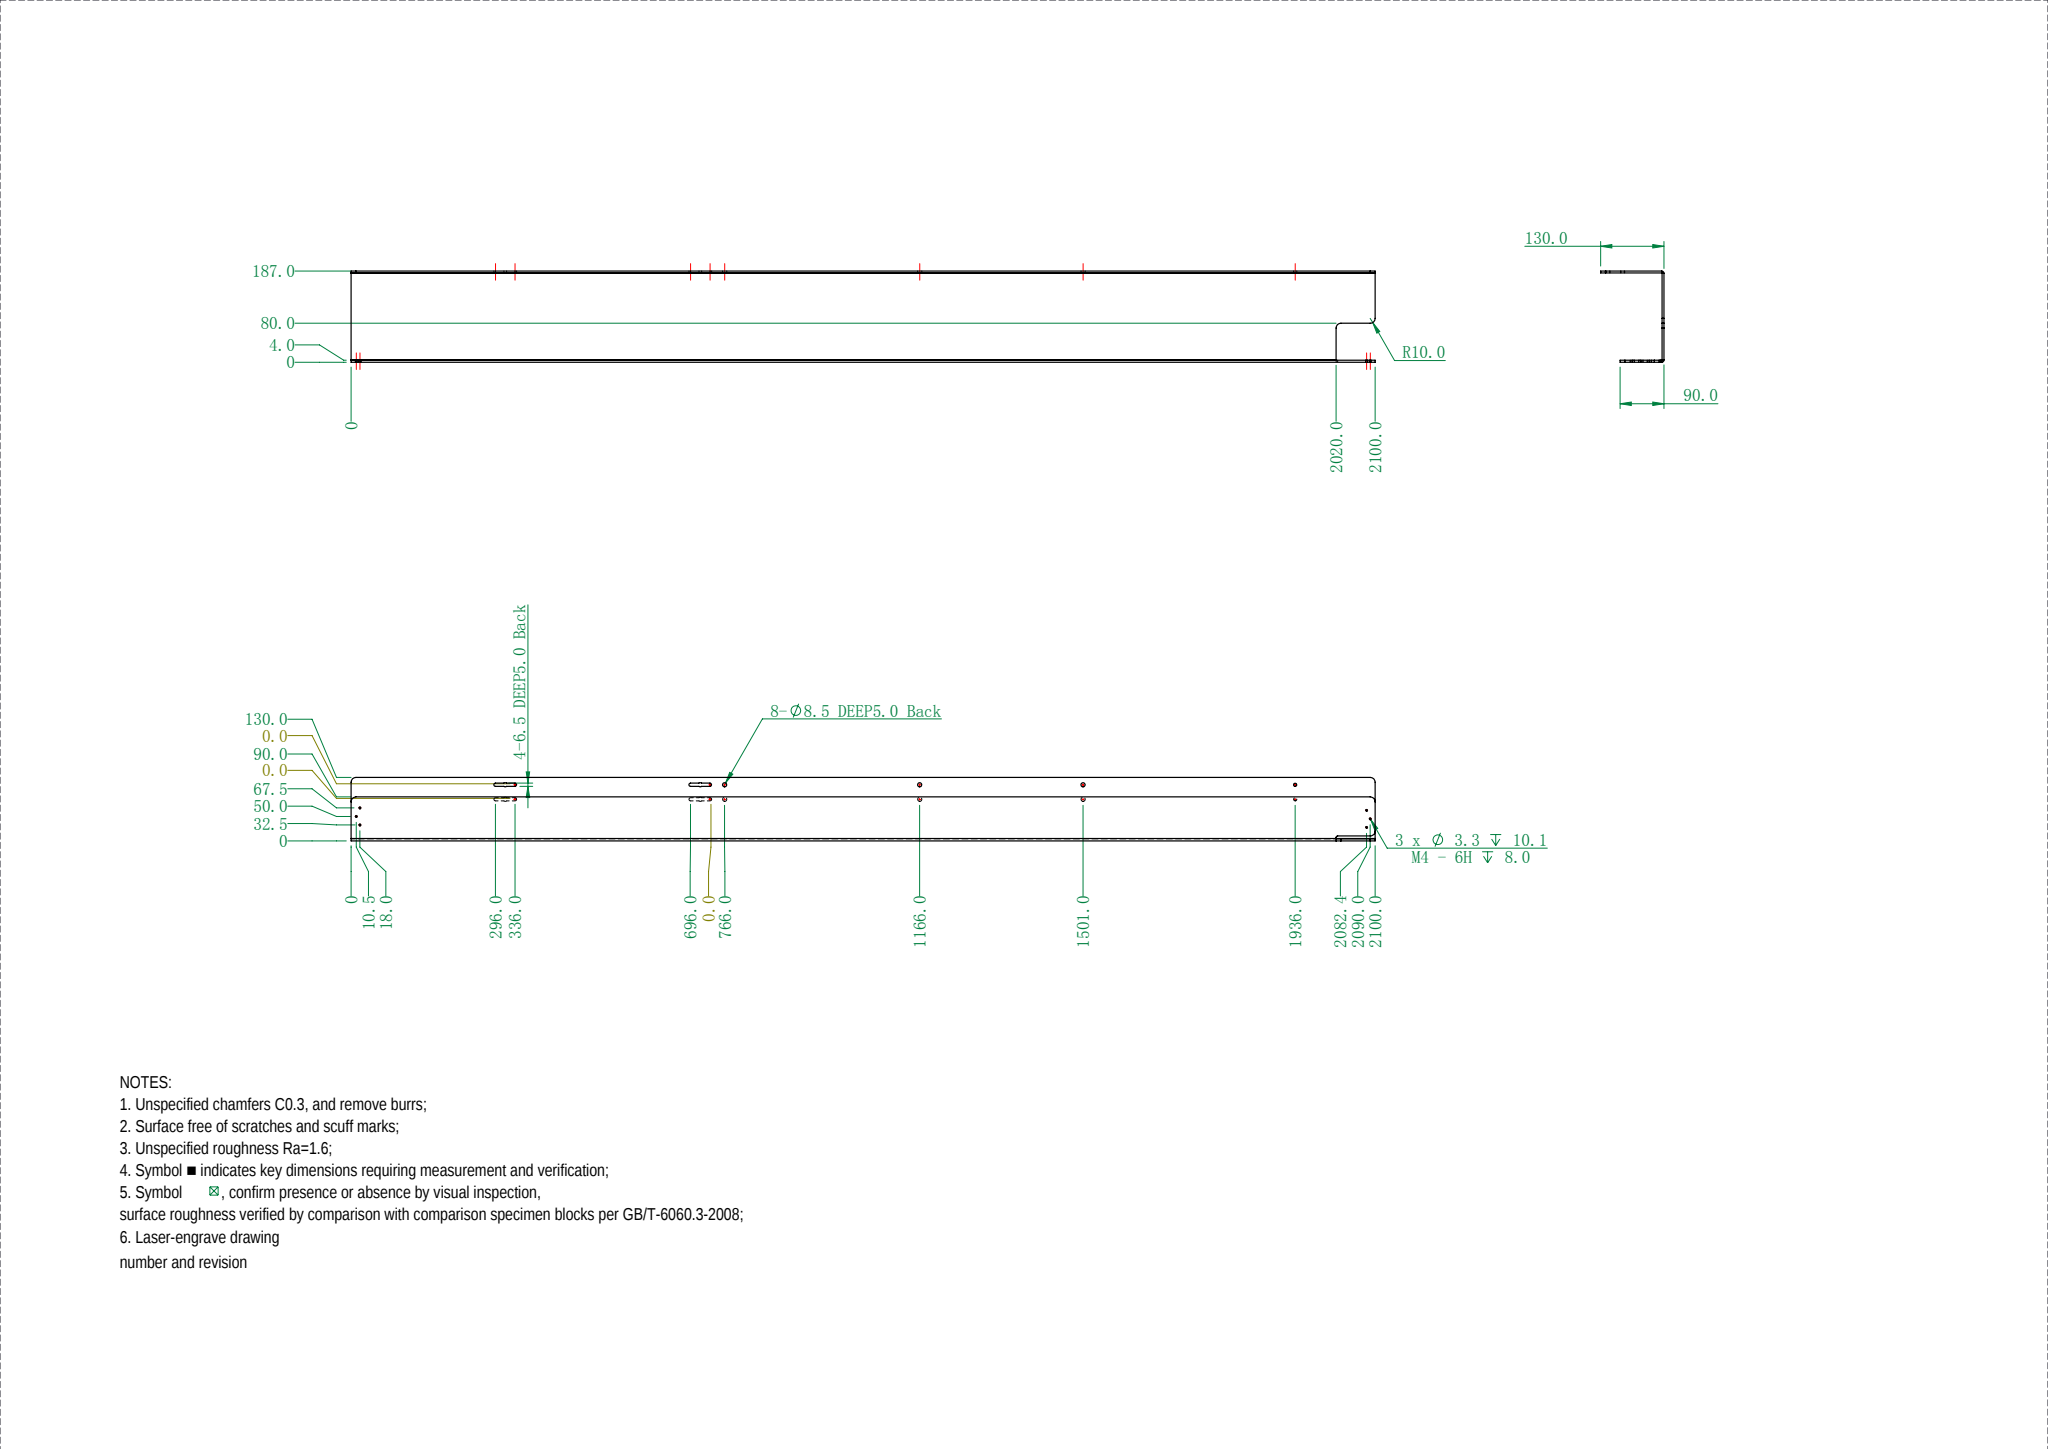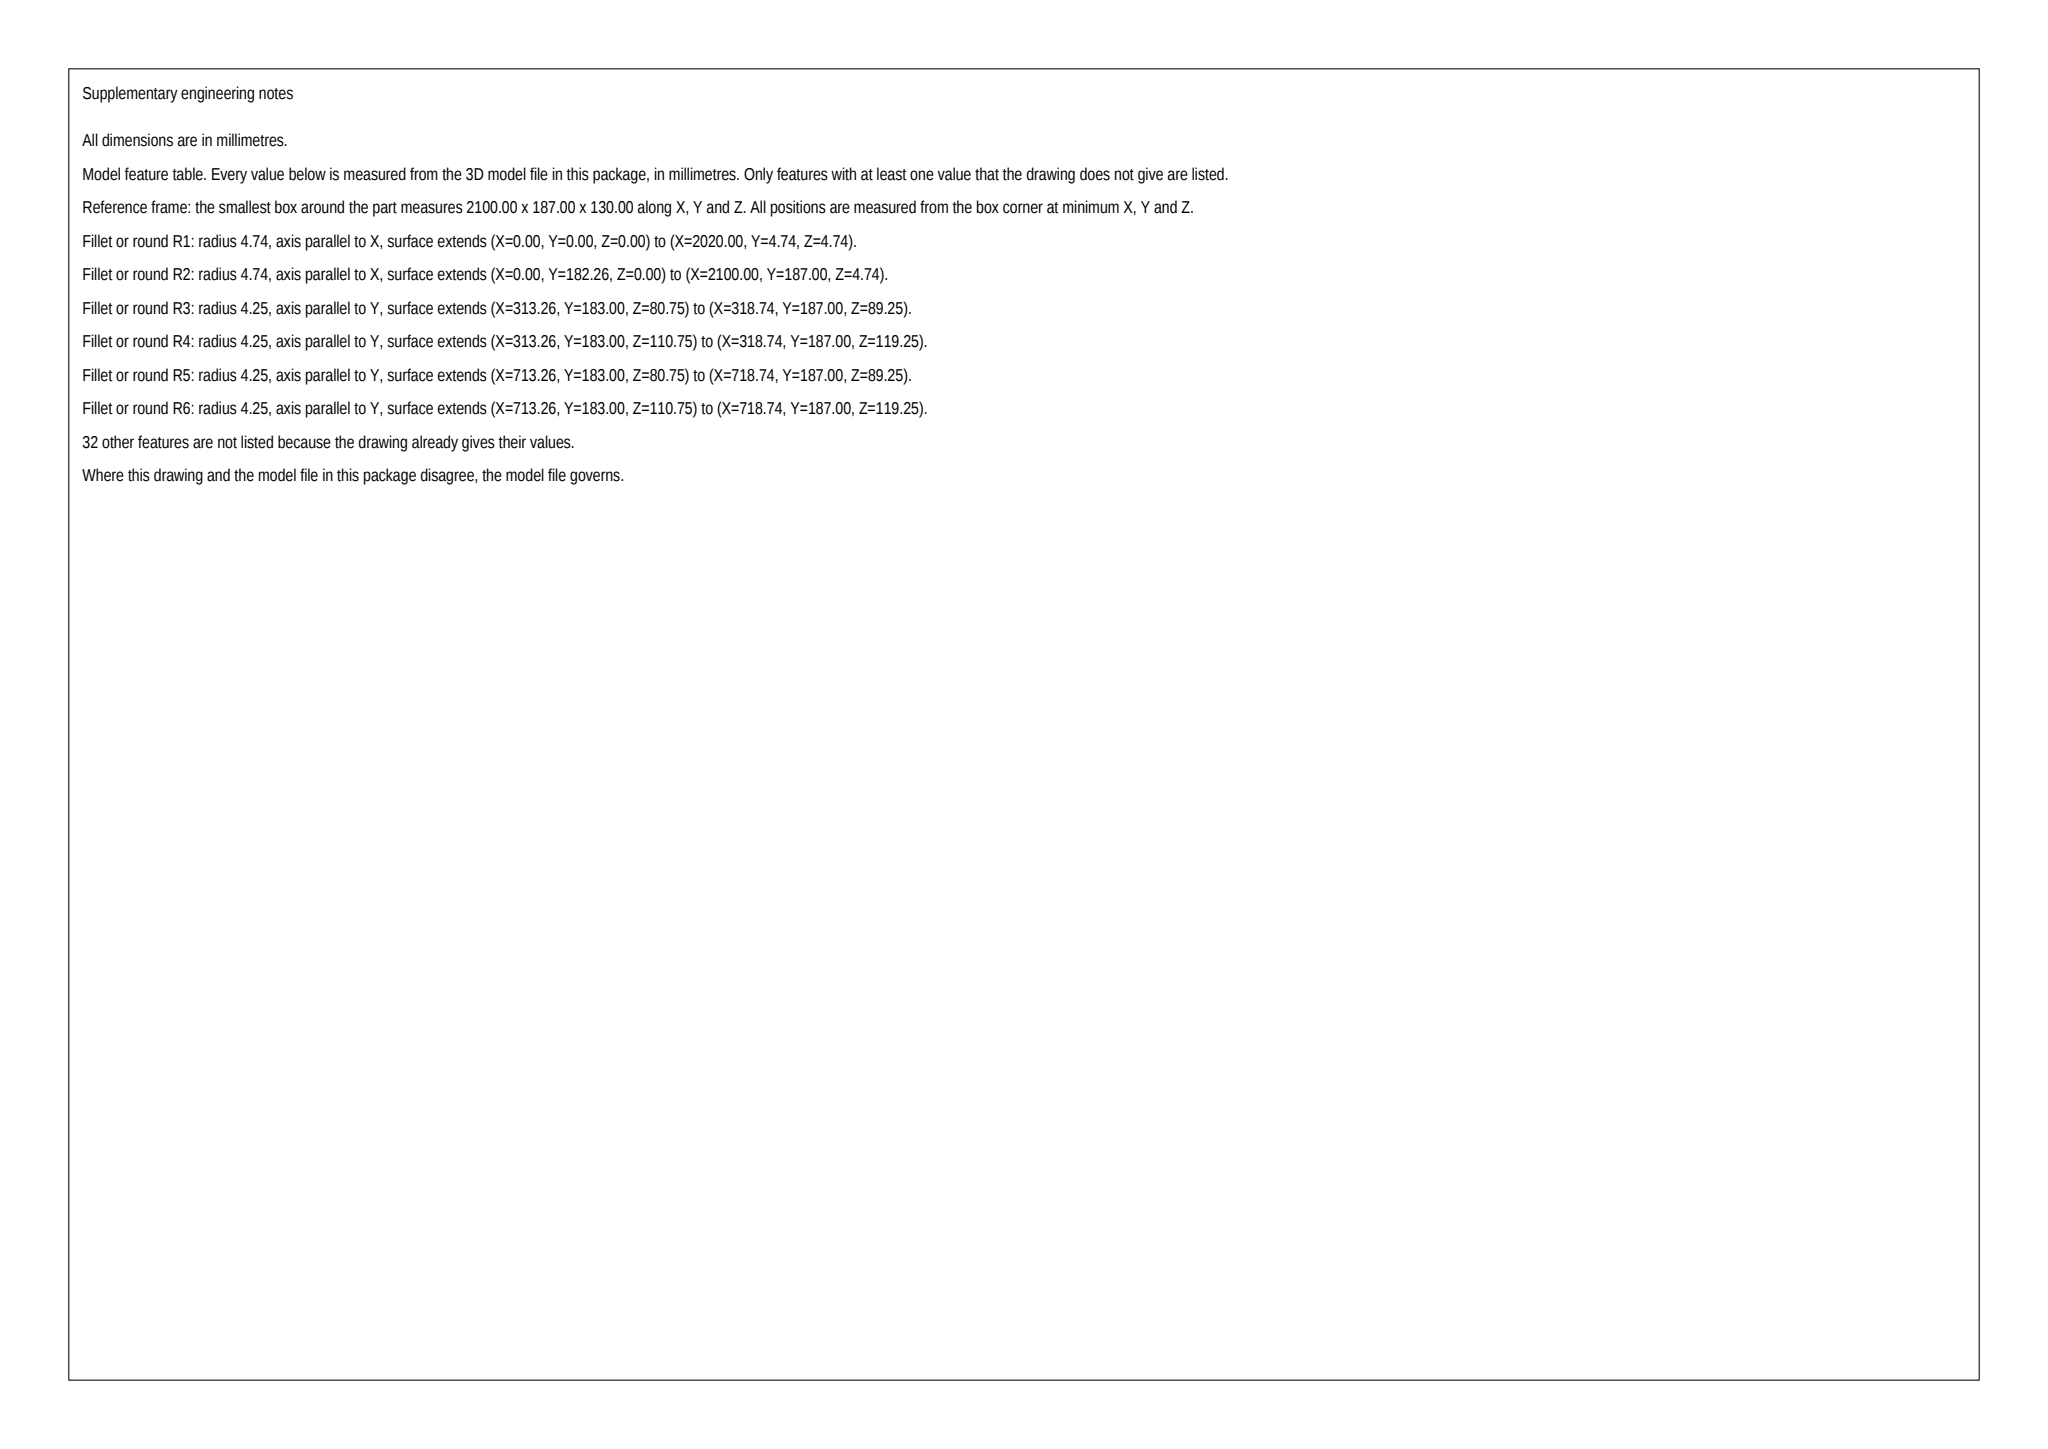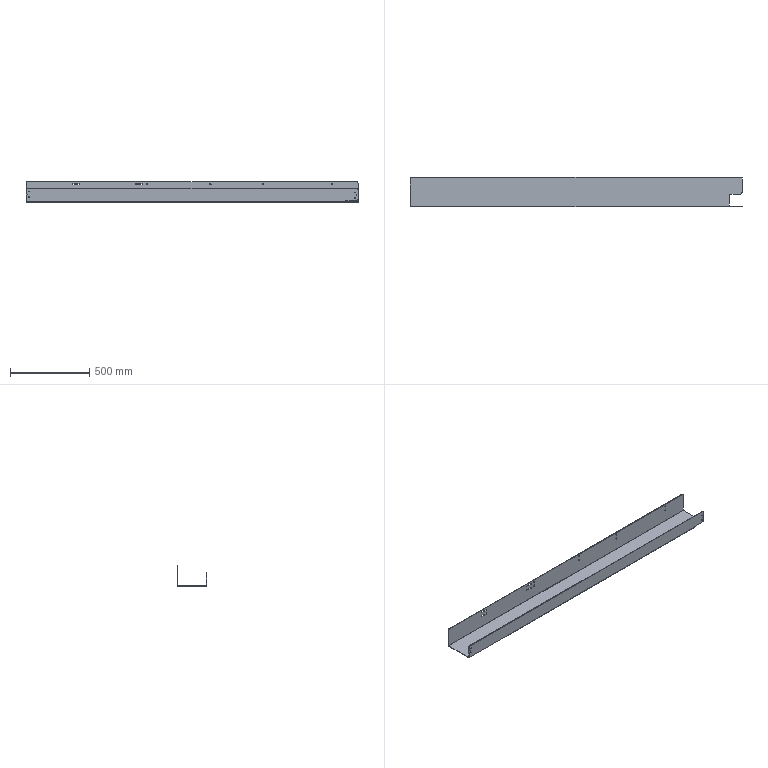Part | SolidWorks | mm | 1 solid | 98 faces | box 2100 x 187 x 130 mm | volume 3297658 mm3 | cylinder 60 | plane 38 | commonest cylinder face diameters 8.5 x24 6.5 x12 3.3 x12 20 x7 9.473 x2 1.473 x2 6 x1